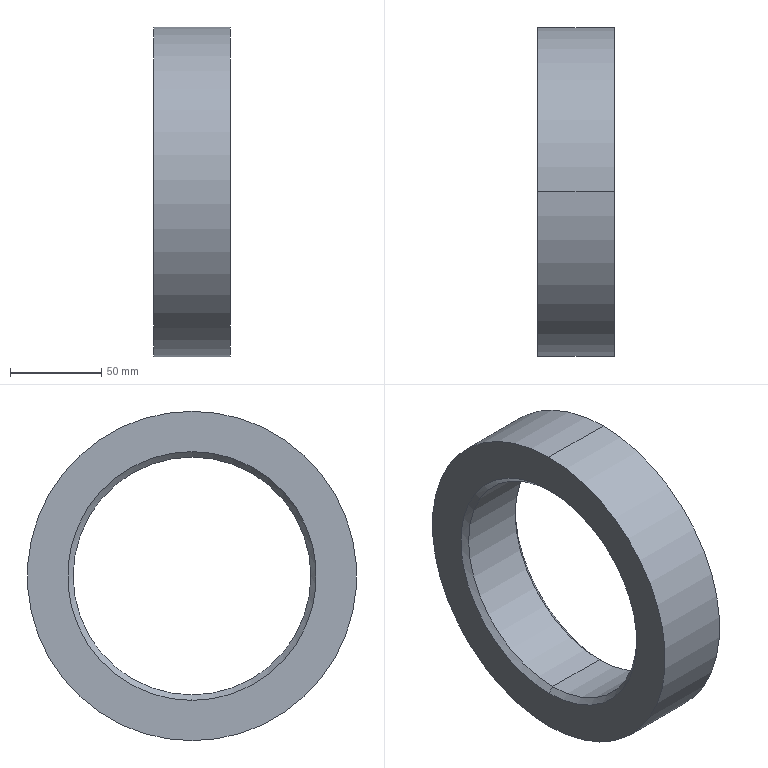Component | SolidWorks | THK-A1009DriveWheelRoundPlate-1 | 1 solid | 10 faces | box 42 x 180 x 180 mm | volume 507562 mm3 | cone 4 | cylinder 4 | plane 2 | commonest cylinder face diameters 130 x2 180 x2 | material 45
build123d program:
from build123d import *

# Parameters (mm, degrees)
SKETCH1_R           = 90
BOSS_EXTRUDE1_DEPTH = 21
SKETCH2_R           = 65
CUT_EXTRUDE1_DEPTH  = 135.03
CHAMFER1_SIZE       = 3


with BuildPart() as part:
    # Sketch1 → Boss-Extrude1 (new, symmetric)
    with BuildSketch(Plane(origin=(0, 0, 0), x_dir=(0, 0, -1), z_dir=(1, 0, 0))):
        with Locations(Location((0, 0, 0), (0, 0, 180))):
            Circle(SKETCH1_R)
    extrude(amount=BOSS_EXTRUDE1_DEPTH, both=True)

    # Sketch2 → Cut-Extrude1 (cut, through all)
    with BuildSketch(Plane(origin=(21, 0, 0), x_dir=(0, 0, -1), z_dir=(1, 0, 0))):
        Circle(SKETCH2_R)
    extrude(amount=-CUT_EXTRUDE1_DEPTH, mode=Mode.SUBTRACT)

    # Chamfer1
    chamfer1_edges = [part.edges().sort_by_distance(p)[0] for p in [
        (-21, 0, 65),
        (21, 0, 65),
    ]]
    chamfer(chamfer1_edges, length=CHAMFER1_SIZE)


solid = part.part

# Placed as in the assembly
solid = solid.moved(Location((76, -5, 191), (0, 0, 0)))
STEP:
#1=COLOUR_RGB('',0.7922,0.8196,0.9333);
#2=FILL_AREA_STYLE_COLOUR('',#1);
#3=FILL_AREA_STYLE('',(#2));
#4=SURFACE_STYLE_FILL_AREA(#3);
#5=SURFACE_SIDE_STYLE('',(#4));
#6=SURFACE_STYLE_USAGE(.BOTH.,#5);
#7=PRESENTATION_STYLE_ASSIGNMENT((#6));
#8=CARTESIAN_POINT('',(3.701,-0.1969,10.079));
#9=VERTEX_POINT('',#8);
#10=CARTESIAN_POINT('',(3.701,-0.1969,4.961));
#11=VERTEX_POINT('',#10);
#12=CARTESIAN_POINT('',(3.701,-0.1969,7.52));
#13=DIRECTION('',(1.,0.,0.));
#14=DIRECTION('',(0.,0.,-1.));
#15=AXIS2_PLACEMENT_3D('',#12,#13,#14);
#16=CIRCLE('',#15,2.559);
#17=EDGE_CURVE('',#9,#11,#16,.T.);
#18=ORIENTED_EDGE('',*,*,#17,.F.);
#19=CARTESIAN_POINT('',(3.819,-0.1969,10.197));
#20=VERTEX_POINT('',#19);
#21=CARTESIAN_POINT('',(3.701,-0.1969,10.079));
#22=DIRECTION('',(0.7071,0.,0.7071));
#23=VECTOR('',#22,39.37);
#24=LINE('',#21,#23);
#25=EDGE_CURVE('',#9,#20,#24,.T.);
#26=ORIENTED_EDGE('',*,*,#25,.T.);
#27=CARTESIAN_POINT('',(3.819,-0.1969,4.843));
#28=VERTEX_POINT('',#27);
#29=CARTESIAN_POINT('',(3.819,-0.1969,7.52));
#30=DIRECTION('',(-1.,0.,0.));
#31=DIRECTION('',(0.,0.,-1.));
#32=AXIS2_PLACEMENT_3D('',#29,#30,#31);
#33=CIRCLE('',#32,2.677);
#34=EDGE_CURVE('',#28,#20,#33,.T.);
#35=ORIENTED_EDGE('',*,*,#34,.F.);
#36=CARTESIAN_POINT('',(3.701,-0.1969,4.961));
#37=DIRECTION('',(0.7071,0.,-0.7071));
#38=VECTOR('',#37,39.37);
#39=LINE('',#36,#38);
#40=EDGE_CURVE('',#11,#28,#39,.T.);
#41=ORIENTED_EDGE('',*,*,#40,.F.);
#42=EDGE_LOOP('',(#18,#26,#35,#41));
#43=FACE_OUTER_BOUND('',#42,.T.);
#44=CARTESIAN_POINT('',(3.701,-0.1969,7.52));
#45=DIRECTION('',(1.,0.,0.));
#46=DIRECTION('',(0.,0.,-1.));
#47=AXIS2_PLACEMENT_3D('',#44,#45,#46);
#48=CONICAL_SURFACE('',#47,2.559,0.7854);
#49=ADVANCED_FACE('',(#43),#48,.F.);
#50=CARTESIAN_POINT('',(2.283,-0.1969,4.961));
#51=VERTEX_POINT('',#50);
#52=CARTESIAN_POINT('',(2.283,-0.1969,10.079));
#53=VERTEX_POINT('',#52);
#54=CARTESIAN_POINT('',(2.283,-0.1969,7.52));
#55=DIRECTION('',(-1.,0.,-0.));
#56=DIRECTION('',(0.,0.,-1.));
#57=AXIS2_PLACEMENT_3D('',#54,#55,#56);
#58=CIRCLE('',#57,2.559);
#59=EDGE_CURVE('',#51,#53,#58,.T.);
#60=ORIENTED_EDGE('',*,*,#59,.F.);
#61=CARTESIAN_POINT('',(2.165,-0.1969,4.843));
#62=VERTEX_POINT('',#61);
#63=CARTESIAN_POINT('',(2.165,-0.1969,4.843));
#64=DIRECTION('',(-0.7071,0.,-0.7071));
#65=VECTOR('',#64,39.37);
#66=LINE('',#63,#65);
#67=EDGE_CURVE('',#51,#62,#66,.T.);
#68=ORIENTED_EDGE('',*,*,#67,.T.);
#69=CARTESIAN_POINT('',(2.165,-0.1969,10.197));
#70=VERTEX_POINT('',#69);
#71=CARTESIAN_POINT('',(2.165,-0.1969,7.52));
#72=DIRECTION('',(1.,0.,0.));
#73=DIRECTION('',(0.,0.,-1.));
#74=AXIS2_PLACEMENT_3D('',#71,#72,#73);
#75=CIRCLE('',#74,2.677);
#76=EDGE_CURVE('',#70,#62,#75,.T.);
#77=ORIENTED_EDGE('',*,*,#76,.F.);
#78=CARTESIAN_POINT('',(2.165,-0.1969,10.197));
#79=DIRECTION('',(-0.7071,0.,0.7071));
#80=VECTOR('',#79,39.37);
#81=LINE('',#78,#80);
#82=EDGE_CURVE('',#53,#70,#81,.T.);
#83=ORIENTED_EDGE('',*,*,#82,.F.);
#84=EDGE_LOOP('',(#60,#68,#77,#83));
#85=FACE_OUTER_BOUND('',#84,.T.);
#86=CARTESIAN_POINT('',(2.165,-0.1969,7.52));
#87=DIRECTION('',(-1.,0.,-0.));
#88=DIRECTION('',(-0.,0.,1.));
#89=AXIS2_PLACEMENT_3D('',#86,#87,#88);
#90=CONICAL_SURFACE('',#89,2.677,0.7854);
#91=ADVANCED_FACE('',(#85),#90,.F.);
#92=ORIENTED_EDGE('',*,*,#59,.T.);
#93=CARTESIAN_POINT('',(2.165,-0.1969,10.079));
#94=DIRECTION('',(1.,0.,0.));
#95=VECTOR('',#94,39.37);
#96=LINE('',#93,#95);
#97=EDGE_CURVE('',#53,#9,#96,.T.);
#98=ORIENTED_EDGE('',*,*,#97,.T.);
#99=ORIENTED_EDGE('',*,*,#17,.T.);
#100=CARTESIAN_POINT('',(2.165,-0.1969,4.961));
#101=DIRECTION('',(1.,0.,0.));
#102=VECTOR('',#101,39.37);
#103=LINE('',#100,#102);
#104=EDGE_CURVE('',#51,#11,#103,.T.);
#105=ORIENTED_EDGE('',*,*,#104,.F.);
#106=EDGE_LOOP('',(#92,#98,#99,#105));
#107=FACE_OUTER_BOUND('',#106,.T.);
#108=CARTESIAN_POINT('',(2.165,-0.1969,7.52));
#109=DIRECTION('',(1.,0.,0.));
#110=DIRECTION('',(0.,0.,-1.));
#111=AXIS2_PLACEMENT_3D('',#108,#109,#110);
#112=CYLINDRICAL_SURFACE('',#111,2.559);
#113=ADVANCED_FACE('',(#107),#112,.F.);
#114=CARTESIAN_POINT('',(3.819,-0.1969,3.976));
#115=VERTEX_POINT('',#114);
#116=CARTESIAN_POINT('',(3.819,-0.1969,11.063));
#117=VERTEX_POINT('',#116);
#118=CARTESIAN_POINT('',(3.819,-0.1969,7.52));
#119=DIRECTION('',(1.,0.,0.));
#120=DIRECTION('',(0.,0.,-1.));
#121=AXIS2_PLACEMENT_3D('',#118,#119,#120);
#122=CIRCLE('',#121,3.543);
#123=EDGE_CURVE('',#115,#117,#122,.T.);
#124=ORIENTED_EDGE('',*,*,#123,.F.);
#125=CARTESIAN_POINT('',(2.165,-0.1969,3.976));
#126=VERTEX_POINT('',#125);
#127=CARTESIAN_POINT('',(3.819,-0.1969,3.976));
#128=DIRECTION('',(-1.,0.,0.));
#129=VECTOR('',#128,39.37);
#130=LINE('',#127,#129);
#131=EDGE_CURVE('',#115,#126,#130,.T.);
#132=ORIENTED_EDGE('',*,*,#131,.T.);
#133=CARTESIAN_POINT('',(2.165,-0.1969,11.063));
#134=VERTEX_POINT('',#133);
#135=CARTESIAN_POINT('',(2.165,-0.1969,7.52));
#136=DIRECTION('',(1.,0.,0.));
#137=DIRECTION('',(0.,0.,-1.));
#138=AXIS2_PLACEMENT_3D('',#135,#136,#137);
#139=CIRCLE('',#138,3.543);
#140=EDGE_CURVE('',#126,#134,#139,.T.);
#141=ORIENTED_EDGE('',*,*,#140,.T.);
#142=CARTESIAN_POINT('',(3.819,-0.1969,11.063));
#143=DIRECTION('',(-1.,0.,0.));
#144=VECTOR('',#143,39.37);
#145=LINE('',#142,#144);
#146=EDGE_CURVE('',#117,#134,#145,.T.);
#147=ORIENTED_EDGE('',*,*,#146,.F.);
#148=EDGE_LOOP('',(#124,#132,#141,#147));
#149=FACE_OUTER_BOUND('',#148,.T.);
#150=CARTESIAN_POINT('',(3.819,-0.1969,7.52));
#151=DIRECTION('',(-1.,0.,0.));
#152=DIRECTION('',(0.,0.,1.));
#153=AXIS2_PLACEMENT_3D('',#150,#151,#152);
#154=CYLINDRICAL_SURFACE('',#153,3.543);
#155=ADVANCED_FACE('',(#149),#154,.T.);
#156=ORIENTED_EDGE('',*,*,#131,.F.);
#157=CARTESIAN_POINT('',(3.819,-0.1969,7.52));
#158=DIRECTION('',(1.,0.,0.));
#159=DIRECTION('',(0.,0.,-1.));
#160=AXIS2_PLACEMENT_3D('',#157,#158,#159);
#161=CIRCLE('',#160,3.543);
#162=EDGE_CURVE('',#117,#115,#161,.T.);
#163=ORIENTED_EDGE('',*,*,#162,.F.);
#164=ORIENTED_EDGE('',*,*,#146,.T.);
#165=CARTESIAN_POINT('',(2.165,-0.1969,7.52));
#166=DIRECTION('',(1.,0.,0.));
#167=DIRECTION('',(0.,0.,-1.));
#168=AXIS2_PLACEMENT_3D('',#165,#166,#167);
#169=CIRCLE('',#168,3.543);
#170=EDGE_CURVE('',#134,#126,#169,.T.);
#171=ORIENTED_EDGE('',*,*,#170,.T.);
#172=EDGE_LOOP('',(#156,#163,#164,#171));
#173=FACE_OUTER_BOUND('',#172,.T.);
#174=CARTESIAN_POINT('',(3.819,-0.1969,7.52));
#175=DIRECTION('',(-1.,0.,0.));
#176=DIRECTION('',(0.,0.,1.));
#177=AXIS2_PLACEMENT_3D('',#174,#175,#176);
#178=CYLINDRICAL_SURFACE('',#177,3.543);
#179=ADVANCED_FACE('',(#173),#178,.T.);
#180=ORIENTED_EDGE('',*,*,#34,.T.);
#181=CARTESIAN_POINT('',(3.819,-0.1969,7.52));
#182=DIRECTION('',(-1.,0.,0.));
#183=DIRECTION('',(0.,0.,-1.));
#184=AXIS2_PLACEMENT_3D('',#181,#182,#183);
#185=CIRCLE('',#184,2.677);
#186=EDGE_CURVE('',#20,#28,#185,.T.);
#187=ORIENTED_EDGE('',*,*,#186,.T.);
#188=EDGE_LOOP('',(#180,#187));
#189=FACE_BOUND('',#188,.T.);
#190=ORIENTED_EDGE('',*,*,#162,.T.);
#191=ORIENTED_EDGE('',*,*,#123,.T.);
#192=EDGE_LOOP('',(#190,#191));
#193=FACE_OUTER_BOUND('',#192,.T.);
#194=CARTESIAN_POINT('',(3.819,-0.1969,7.52));
#195=DIRECTION('',(1.,0.,0.));
#196=DIRECTION('',(0.,0.,-1.));
#197=AXIS2_PLACEMENT_3D('',#194,#195,#196);
#198=PLANE('',#197);
#199=ADVANCED_FACE('',(#189,#193),#198,.T.);
#200=ORIENTED_EDGE('',*,*,#76,.T.);
#201=CARTESIAN_POINT('',(2.165,-0.1969,7.52));
#202=DIRECTION('',(1.,0.,0.));
#203=DIRECTION('',(0.,0.,-1.));
#204=AXIS2_PLACEMENT_3D('',#201,#202,#203);
#205=CIRCLE('',#204,2.677);
#206=EDGE_CURVE('',#62,#70,#205,.T.);
#207=ORIENTED_EDGE('',*,*,#206,.T.);
#208=EDGE_LOOP('',(#200,#207));
#209=FACE_BOUND('',#208,.T.);
#210=ORIENTED_EDGE('',*,*,#170,.F.);
#211=ORIENTED_EDGE('',*,*,#140,.F.);
#212=EDGE_LOOP('',(#210,#211));
#213=FACE_OUTER_BOUND('',#212,.T.);
#214=CARTESIAN_POINT('',(2.165,-0.1969,7.52));
#215=DIRECTION('',(1.,0.,0.));
#216=DIRECTION('',(0.,0.,-1.));
#217=AXIS2_PLACEMENT_3D('',#214,#215,#216);
#218=PLANE('',#217);
#219=ADVANCED_FACE('',(#209,#213),#218,.F.);
#220=ORIENTED_EDGE('',*,*,#97,.F.);
#221=CARTESIAN_POINT('',(2.283,-0.1969,7.52));
#222=DIRECTION('',(-1.,0.,-0.));
#223=DIRECTION('',(0.,0.,-1.));
#224=AXIS2_PLACEMENT_3D('',#221,#222,#223);
#225=CIRCLE('',#224,2.559);
#226=EDGE_CURVE('',#53,#51,#225,.T.);
#227=ORIENTED_EDGE('',*,*,#226,.T.);
#228=ORIENTED_EDGE('',*,*,#104,.T.);
#229=CARTESIAN_POINT('',(3.701,-0.1969,7.52));
#230=DIRECTION('',(1.,0.,0.));
#231=DIRECTION('',(0.,0.,-1.));
#232=AXIS2_PLACEMENT_3D('',#229,#230,#231);
#233=CIRCLE('',#232,2.559);
#234=EDGE_CURVE('',#11,#9,#233,.T.);
#235=ORIENTED_EDGE('',*,*,#234,.T.);
#236=EDGE_LOOP('',(#220,#227,#228,#235));
#237=FACE_OUTER_BOUND('',#236,.T.);
#238=CARTESIAN_POINT('',(2.165,-0.1969,7.52));
#239=DIRECTION('',(1.,0.,0.));
#240=DIRECTION('',(0.,0.,-1.));
#241=AXIS2_PLACEMENT_3D('',#238,#239,#240);
#242=CYLINDRICAL_SURFACE('',#241,2.559);
#243=ADVANCED_FACE('',(#237),#242,.F.);
#244=ORIENTED_EDGE('',*,*,#67,.F.);
#245=ORIENTED_EDGE('',*,*,#226,.F.);
#246=ORIENTED_EDGE('',*,*,#82,.T.);
#247=ORIENTED_EDGE('',*,*,#206,.F.);
#248=EDGE_LOOP('',(#244,#245,#246,#247));
#249=FACE_OUTER_BOUND('',#248,.T.);
#250=CARTESIAN_POINT('',(2.165,-0.1969,7.52));
#251=DIRECTION('',(-1.,0.,-0.));
#252=DIRECTION('',(-0.,0.,1.));
#253=AXIS2_PLACEMENT_3D('',#250,#251,#252);
#254=CONICAL_SURFACE('',#253,2.677,0.7854);
#255=ADVANCED_FACE('',(#249),#254,.F.);
#256=ORIENTED_EDGE('',*,*,#25,.F.);
#257=ORIENTED_EDGE('',*,*,#234,.F.);
#258=ORIENTED_EDGE('',*,*,#40,.T.);
#259=ORIENTED_EDGE('',*,*,#186,.F.);
#260=EDGE_LOOP('',(#256,#257,#258,#259));
#261=FACE_OUTER_BOUND('',#260,.T.);
#262=CARTESIAN_POINT('',(3.701,-0.1969,7.52));
#263=DIRECTION('',(1.,0.,0.));
#264=DIRECTION('',(0.,0.,-1.));
#265=AXIS2_PLACEMENT_3D('',#262,#263,#264);
#266=CONICAL_SURFACE('',#265,2.559,0.7854);
#267=ADVANCED_FACE('',(#261),#266,.F.);
#268=CLOSED_SHELL('',(#49,#91,#113,#155,#179,#199,#219,#243,#255,#267));
#269=MANIFOLD_SOLID_BREP('',#268);
#270=STYLED_ITEM('',(#7),#269);
#271=PRESENTATION_LAYER_ASSIGNMENT('','',(#270));
#272=CARTESIAN_POINT('',(0.,0.,0.));
#273=DIRECTION('',(0.,0.,1.));
#274=DIRECTION('',(1.,0.,0.));
#275=AXIS2_PLACEMENT_3D('',#272,#273,#274);
#276=(LENGTH_UNIT()NAMED_UNIT(*)SI_UNIT($,.METRE.));
#277=LENGTH_MEASURE_WITH_UNIT(LENGTH_MEASURE(0.0254),#276);
#278=DIMENSIONAL_EXPONENTS(1.,0.,0.,0.,0.,0.,0.);
#279=(CONVERSION_BASED_UNIT('',#277)LENGTH_UNIT()NAMED_UNIT(#278));
#280=UNCERTAINTY_MEASURE_WITH_UNIT(LENGTH_MEASURE(0.00001),#279,'','');
#281=(NAMED_UNIT(*)PLANE_ANGLE_UNIT()SI_UNIT($,.RADIAN.));
#282=(NAMED_UNIT(*)SI_UNIT($,.STERADIAN.)SOLID_ANGLE_UNIT());
#283=(GEOMETRIC_REPRESENTATION_CONTEXT(3)GLOBAL_UNCERTAINTY_ASSIGNED_CONTEXT((#280))GLOBAL_UNIT_ASSIGNED_CONTEXT((#279,#281,#282))REPRESENTATION_CONTEXT('',''));
#284=ADVANCED_BREP_SHAPE_REPRESENTATION('',(#269,#275),#283);
#285=(LENGTH_UNIT()NAMED_UNIT(*)SI_UNIT($,.METRE.));
#286=LENGTH_MEASURE_WITH_UNIT(LENGTH_MEASURE(0.0254),#285);
#287=DIMENSIONAL_EXPONENTS(1.,0.,0.,0.,0.,0.,0.);
#288=(CONVERSION_BASED_UNIT('',#286)LENGTH_UNIT()NAMED_UNIT(#287));
#289=UNCERTAINTY_MEASURE_WITH_UNIT(LENGTH_MEASURE(0.00001),#288,'','');
#290=(NAMED_UNIT(*)PLANE_ANGLE_UNIT()SI_UNIT($,.RADIAN.));
#291=(NAMED_UNIT(*)SI_UNIT($,.STERADIAN.)SOLID_ANGLE_UNIT());
#292=(GEOMETRIC_REPRESENTATION_CONTEXT(3)GLOBAL_UNCERTAINTY_ASSIGNED_CONTEXT((#289))GLOBAL_UNIT_ASSIGNED_CONTEXT((#288,#290,#291))REPRESENTATION_CONTEXT('',''));
#293=MECHANICAL_DESIGN_GEOMETRIC_PRESENTATION_REPRESENTATION('',(#270),#292);